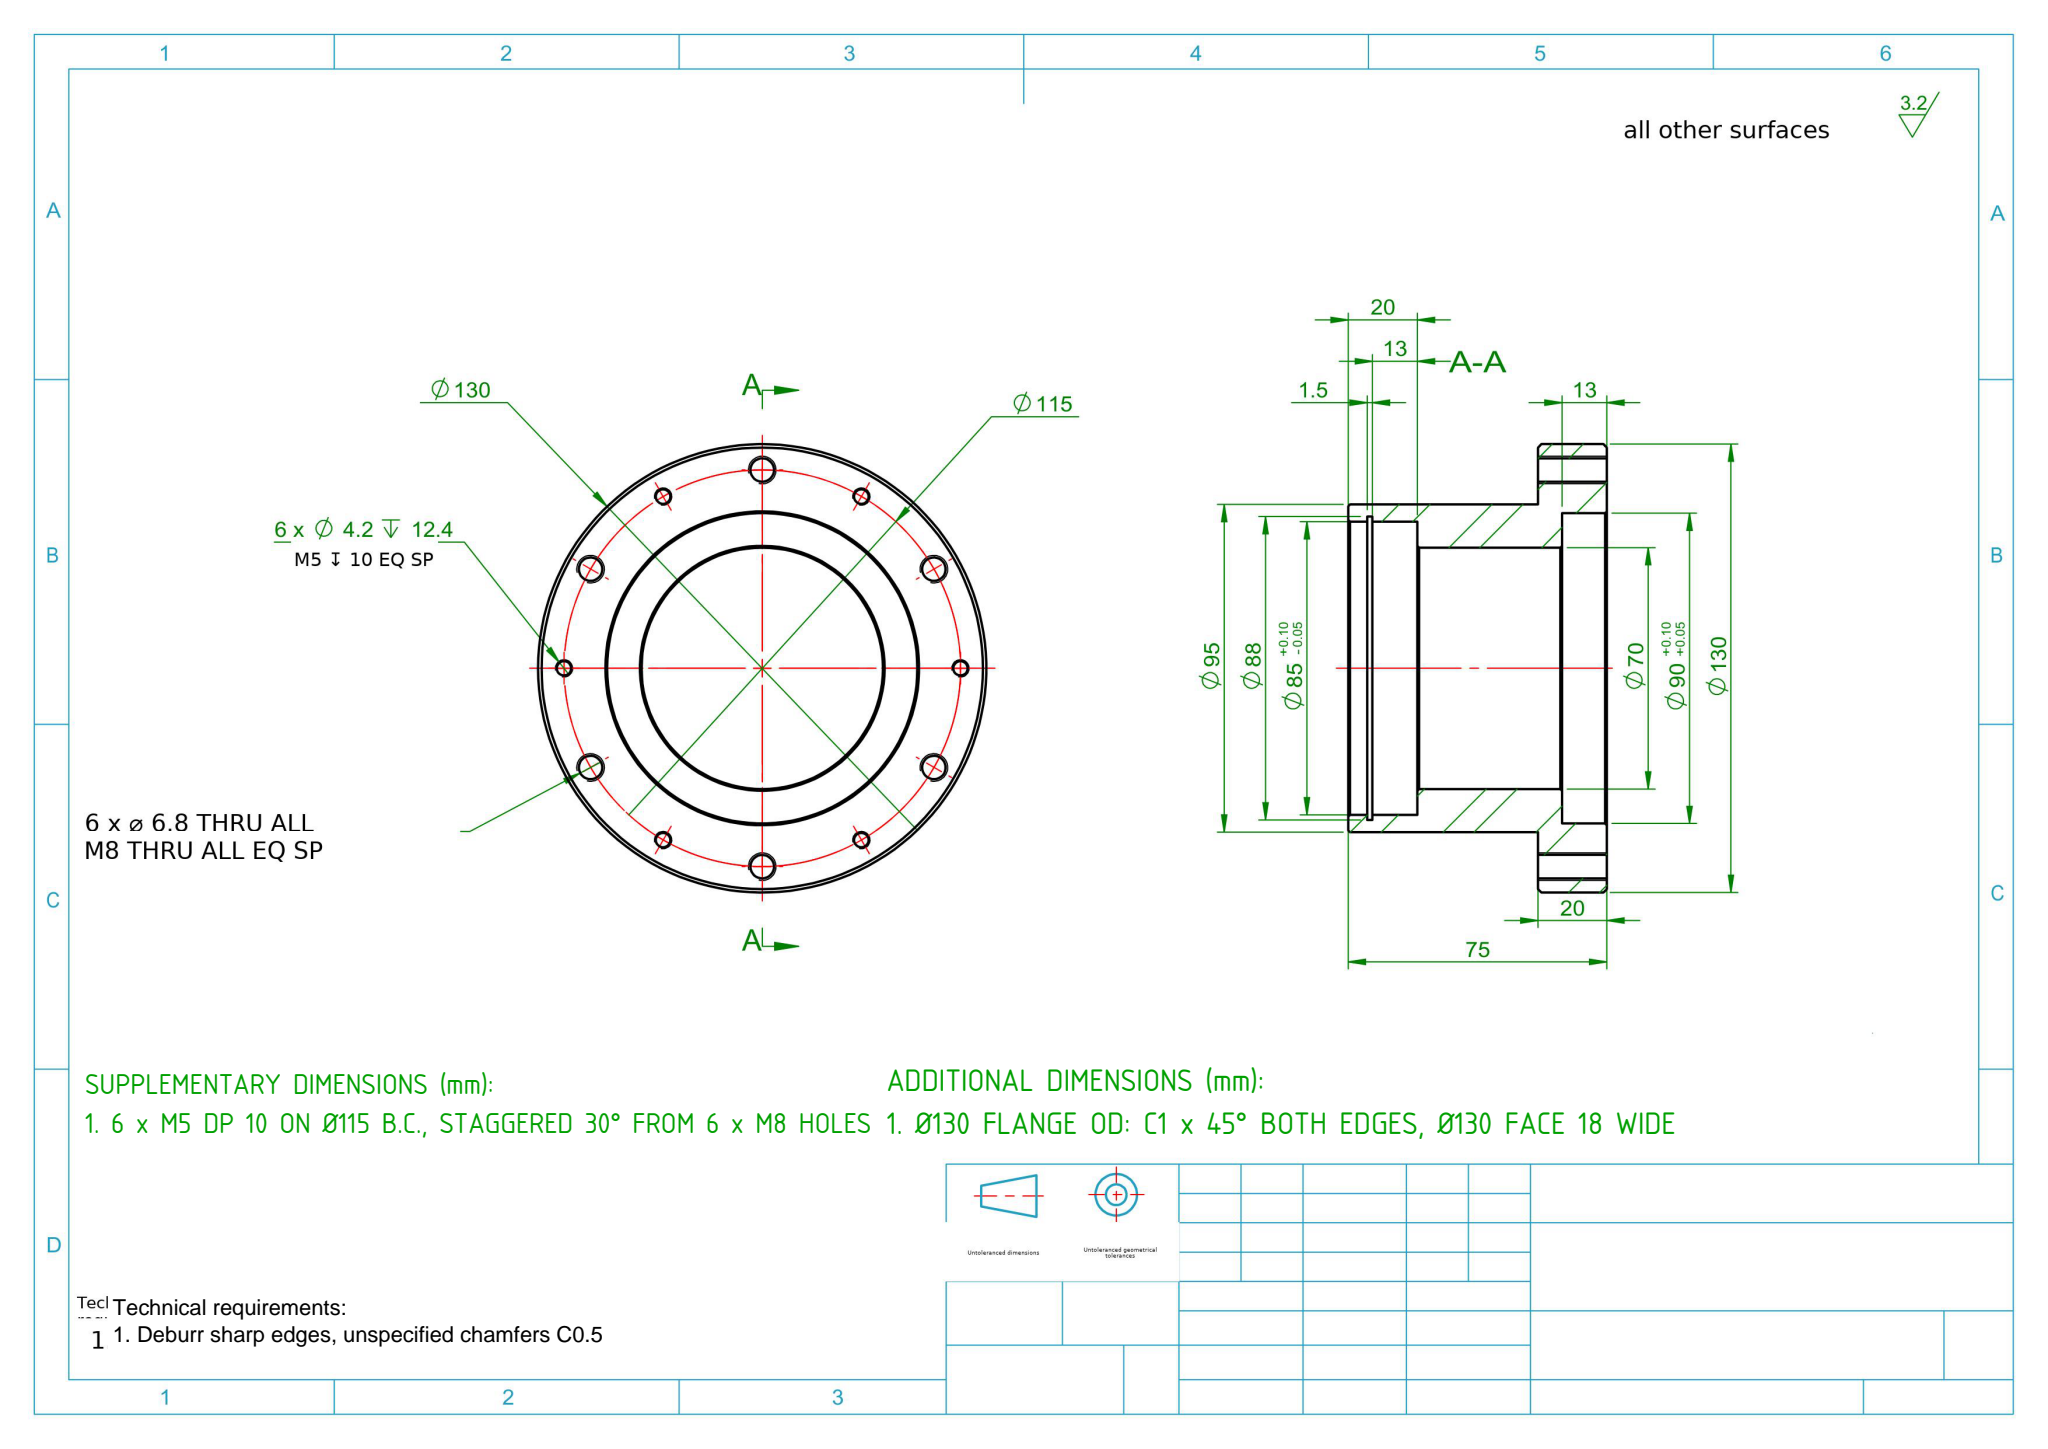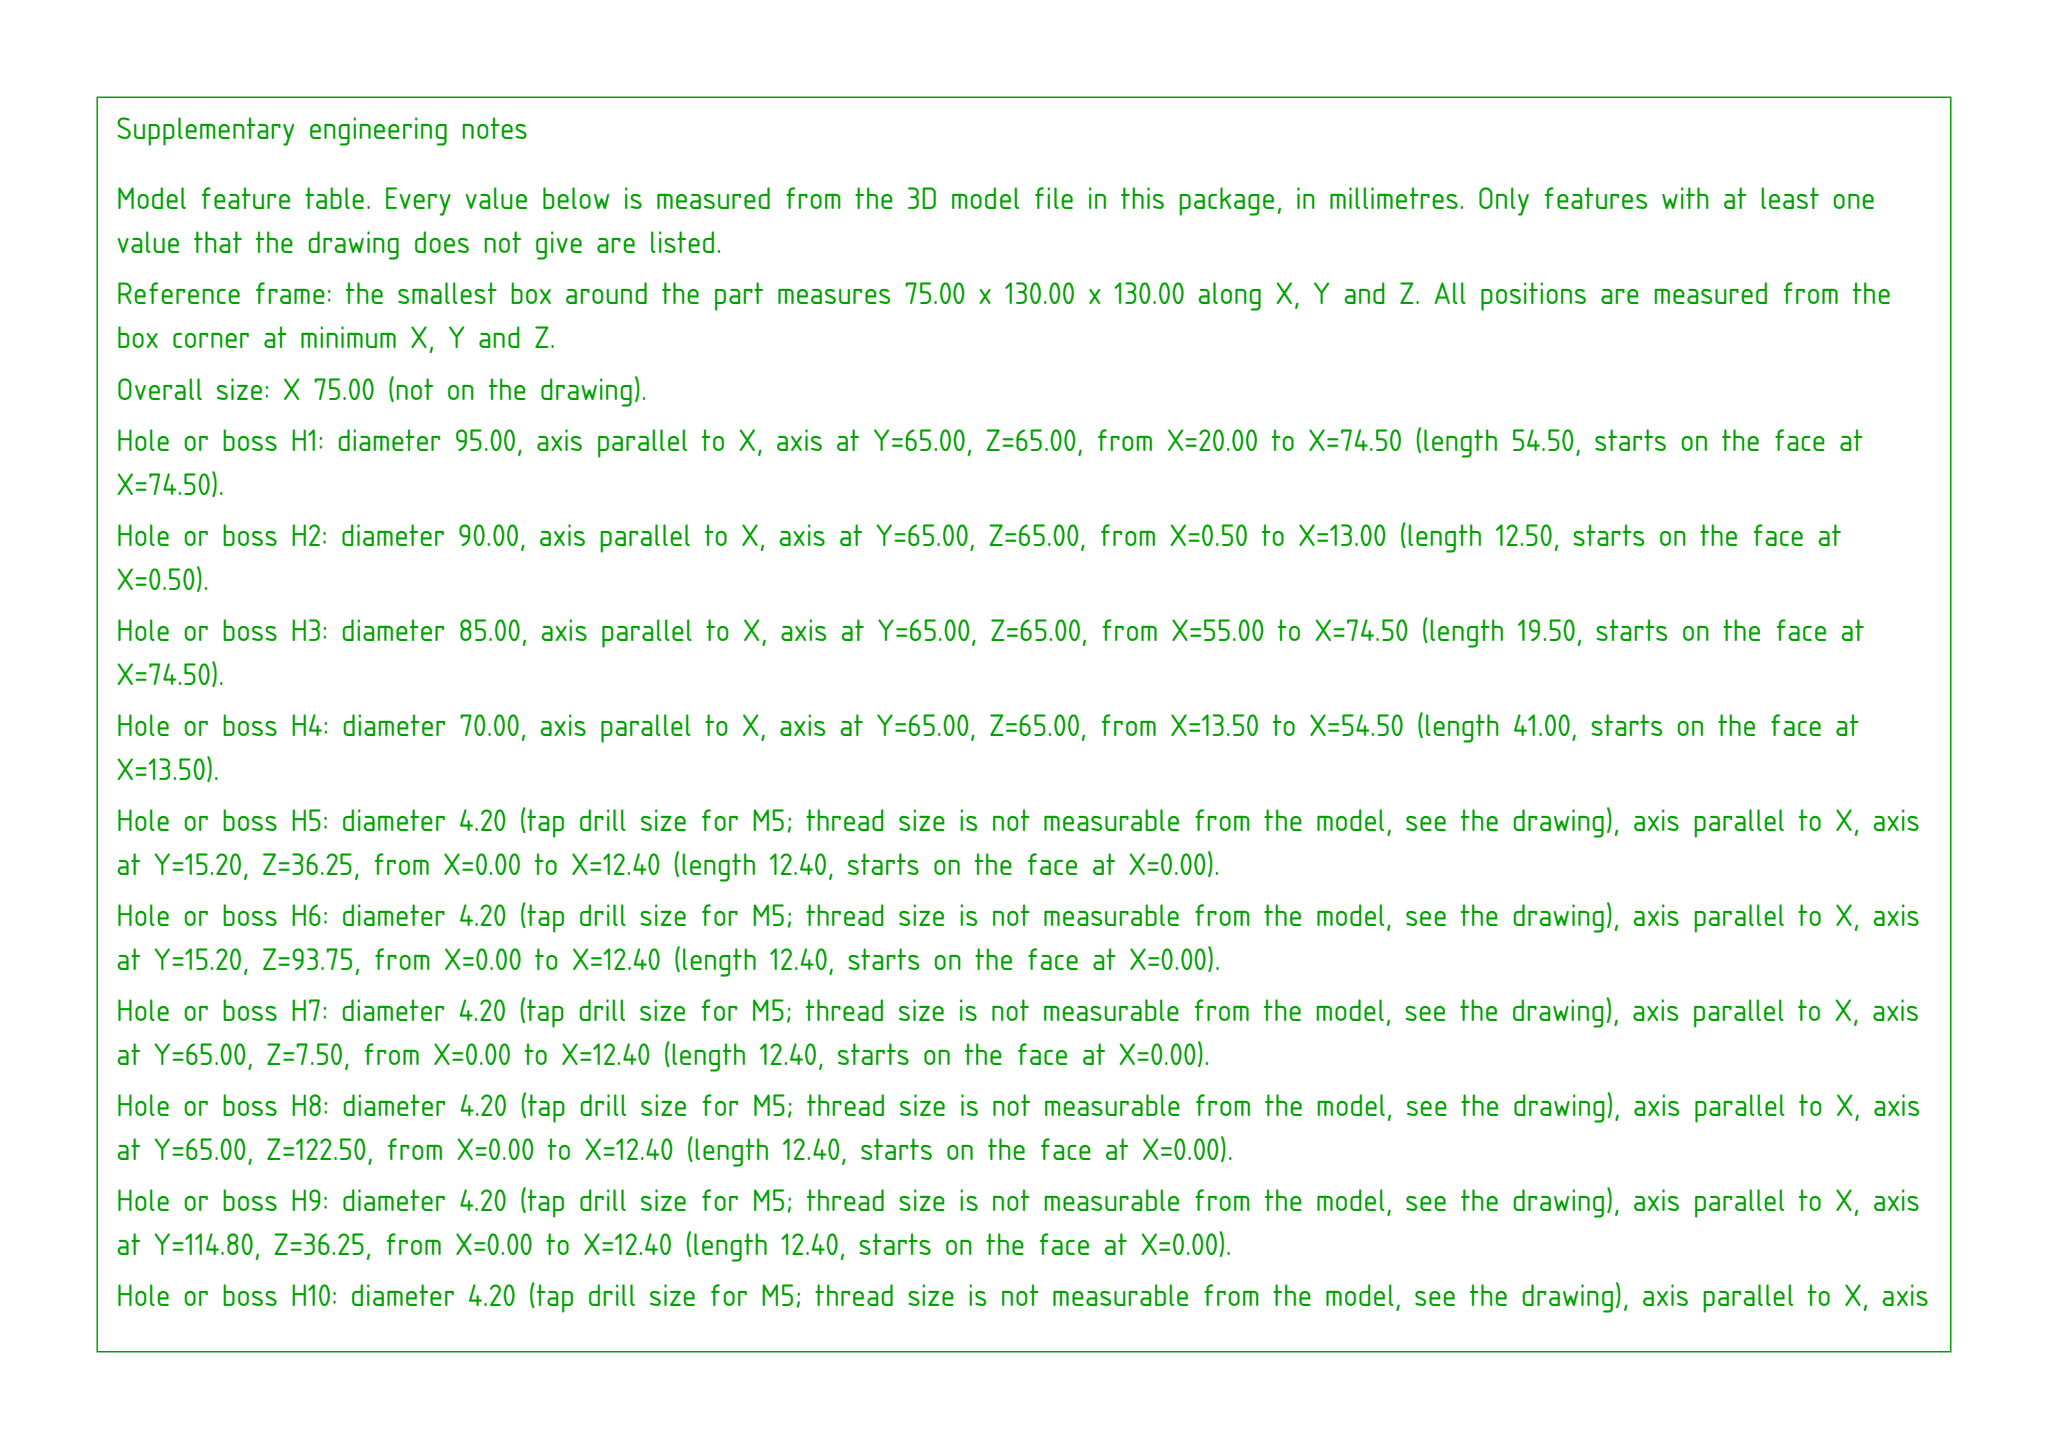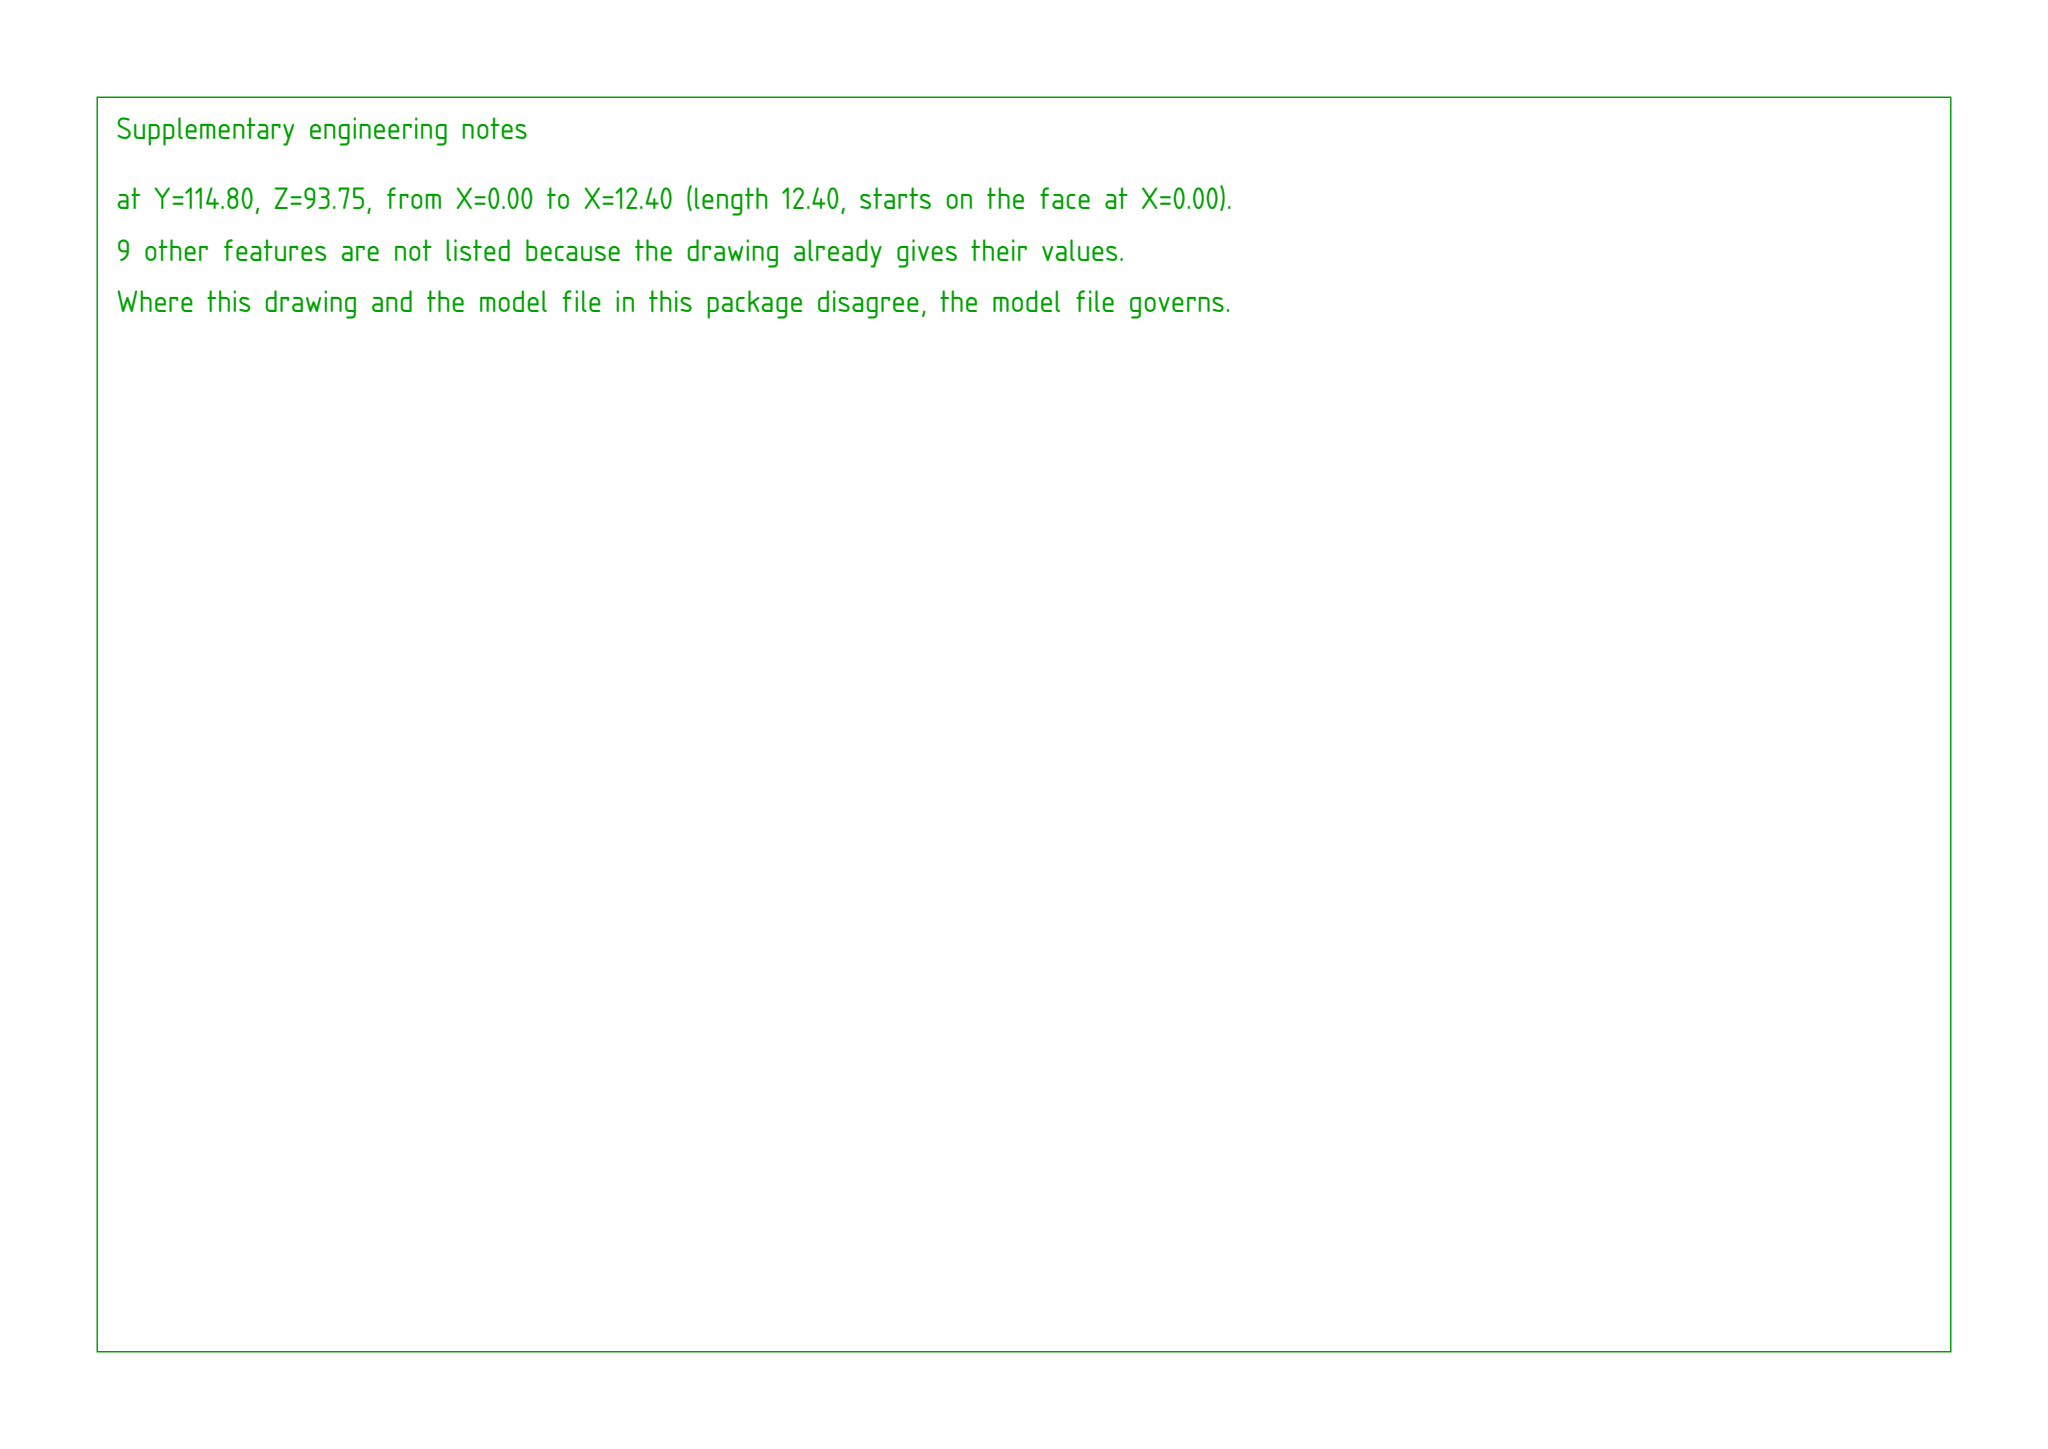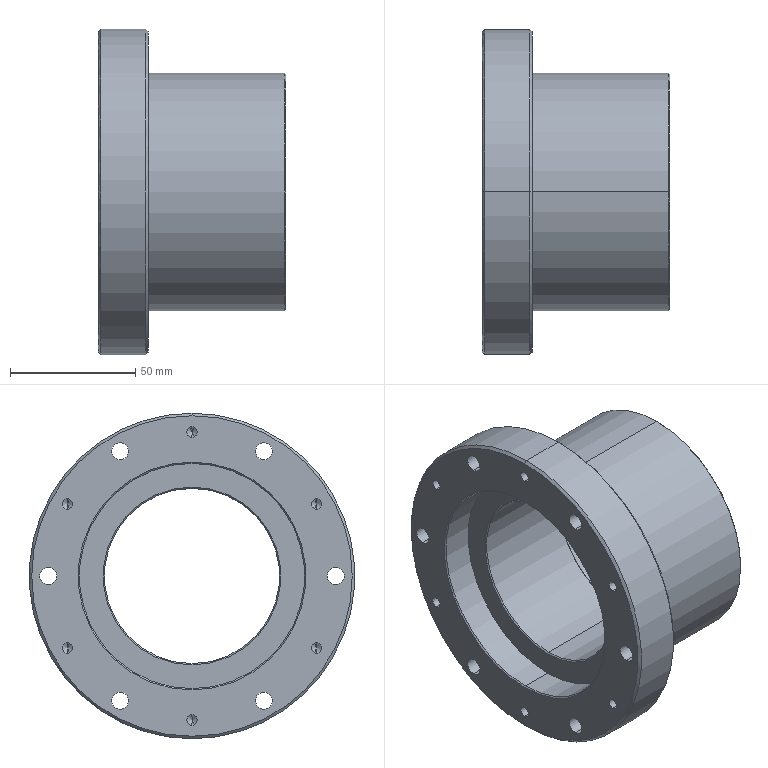Part | SolidWorks | mm | 1 solid | 71 faces | box 75 x 130 x 130 mm | volume 290886 mm3 | cylinder 38 | cone 26 | plane 7 | commonest cylinder face diameters 6.8 x12 4.2 x12 85 x4 88 x2 70 x2 90 x2 95 x2 130 x2
build123d program:
from build123d import *

# Parameters (mm, degrees)
SKETCH1_R             = 65
BOSS_EXTRUDE1_DEPTH   = 20
SKETCH2_R             = 47.5
BOSS_EXTRUDE2_DEPTH   = 55
SKETCH3_R             = 42.5
CUT_EXTRUDE1_DEPTH    = 20
SKETCH4_R             = 45
CUT_EXTRUDE2_DEPTH    = 13
SKETCH5_R             = 35
CUT_EXTRUDE3_DEPTH    = 108.121
CHAMFER1_SIZE         = 1
CHAMFER2_SIZE         = 0.5
M5_TAPPED_HOLE1_D     = 4.2
M5_TAPPED_HOLE1_DEPTH = 12.4
M5_TAPPED_HOLE1_TIP   = 1.262
M8_TAPPED_HOLE1_D     = 6.8
SKETCH11_W            = 1.5
SKETCH11_H            = 1.5


with BuildPart() as part:
    # Sketch1 → Boss-Extrude1 (new body)
    with BuildSketch(Plane(origin=(0, 0, 0), x_dir=(0, 0, -1), z_dir=(1, 0, 0))):
        Circle(SKETCH1_R)
    extrude(amount=BOSS_EXTRUDE1_DEPTH)

    # Sketch2 → Boss-Extrude2 (add)
    with BuildSketch(Plane(origin=(20, 0, 0), x_dir=(0, 0, -1), z_dir=(1, 0, 0))):
        Circle(SKETCH2_R)
    extrude(amount=BOSS_EXTRUDE2_DEPTH)

    # Sketch3 → Cut-Extrude1 (cut)
    with BuildSketch(Plane(origin=(75, 0, 0), x_dir=(0, 0, -1), z_dir=(1, 0, 0))):
        Circle(SKETCH3_R)
    extrude(amount=-CUT_EXTRUDE1_DEPTH, mode=Mode.SUBTRACT)

    # Sketch4 → Cut-Extrude2 (cut)
    with BuildSketch(Plane.ZY):
        Circle(SKETCH4_R)
    extrude(amount=-CUT_EXTRUDE2_DEPTH, mode=Mode.SUBTRACT)

    # Sketch5 → Cut-Extrude3 (cut, through all)
    with BuildSketch(Plane(origin=(55, 0, 0), x_dir=(0, 0, -1), z_dir=(1, 0, 0))):
        Circle(SKETCH5_R)
    extrude(amount=-CUT_EXTRUDE3_DEPTH, mode=Mode.SUBTRACT)

    # Chamfer1
    chamfer1_edges = [part.edges().sort_by_distance(p)[0] for p in [
        (0, 0, 65),
        (20, 0, 65),
    ]]
    chamfer(chamfer1_edges, length=CHAMFER1_SIZE)

    # Chamfer2
    chamfer2_edges = [part.edges().sort_by_distance(p)[0] for p in [
        (75, 0, 42.5),
        (0, 0, -45),
        (13, 0, 35),
        (55, 0, 35),
        (75, 0, 47.5),
    ]]
    chamfer(chamfer2_edges, length=CHAMFER2_SIZE)

    # M5 Tapped Hole1
    with Locations(Plane.ZY):
        with Locations((-57.5, 0), (-28.75, -49.796), (-28.75, 49.796), (28.75, -49.796), (28.75, 49.796), (57.5, 0)):
            Hole(M5_TAPPED_HOLE1_D / 2, depth=M5_TAPPED_HOLE1_DEPTH)
            with Locations((0, 0, -(M5_TAPPED_HOLE1_DEPTH + M5_TAPPED_HOLE1_TIP / 2))):  # 118° drill point
                Cone(0, M5_TAPPED_HOLE1_D / 2, M5_TAPPED_HOLE1_TIP, mode=Mode.SUBTRACT)

    # M8 Tapped Hole1 (through all)
    with Locations(Plane(origin=(20, 0, 0), x_dir=(0, 0, -1), z_dir=(1, 0, 0))):
        with Locations((49.796, 28.75), (49.796, -28.75), (0, 57.5), (-49.796, 28.75), (-49.796, -28.75), (0, -57.5)):
            Hole(M8_TAPPED_HOLE1_D / 2)

    # Sketch11 → Cut-Revolve1 (revolve, cut)
    with BuildSketch(Plane(origin=(0, 0, 0), x_dir=(1, 0, 0), z_dir=(0, 1, 0))):
        with Locations((68.75, 43.25)):
            Rectangle(SKETCH11_W, SKETCH11_H)
    revolve(axis=Axis((0, 0, 0), (1, 0, 0)), mode=Mode.SUBTRACT)


solid = part.part